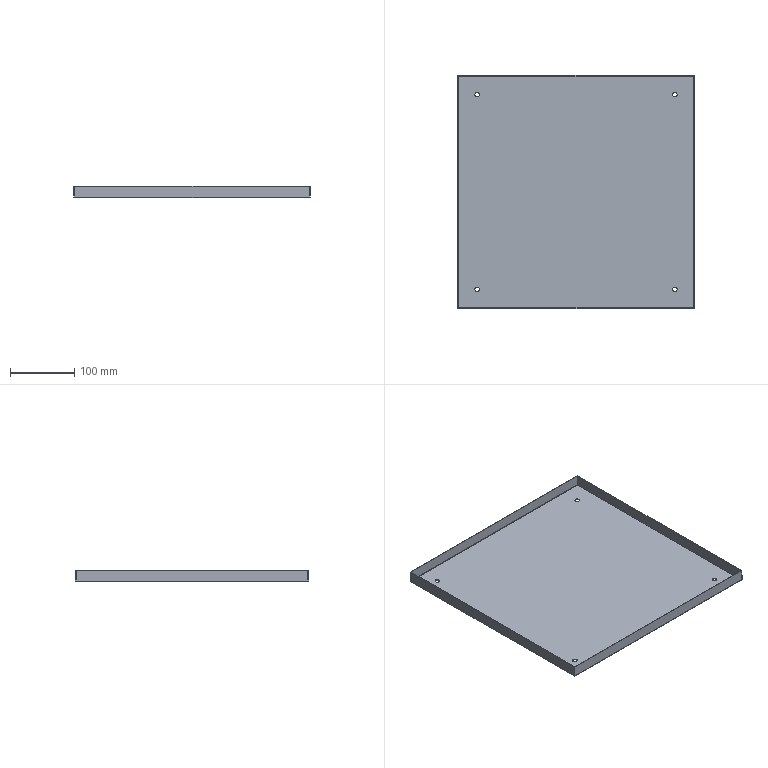Component | SolidWorks | RearPanel-1 | 1 solid | 50 faces | volume 157037 mm3 | plane 34 | cylinder 16 | commonest cylinder face diameters 7 x8 2.2 x4 0.2 x4